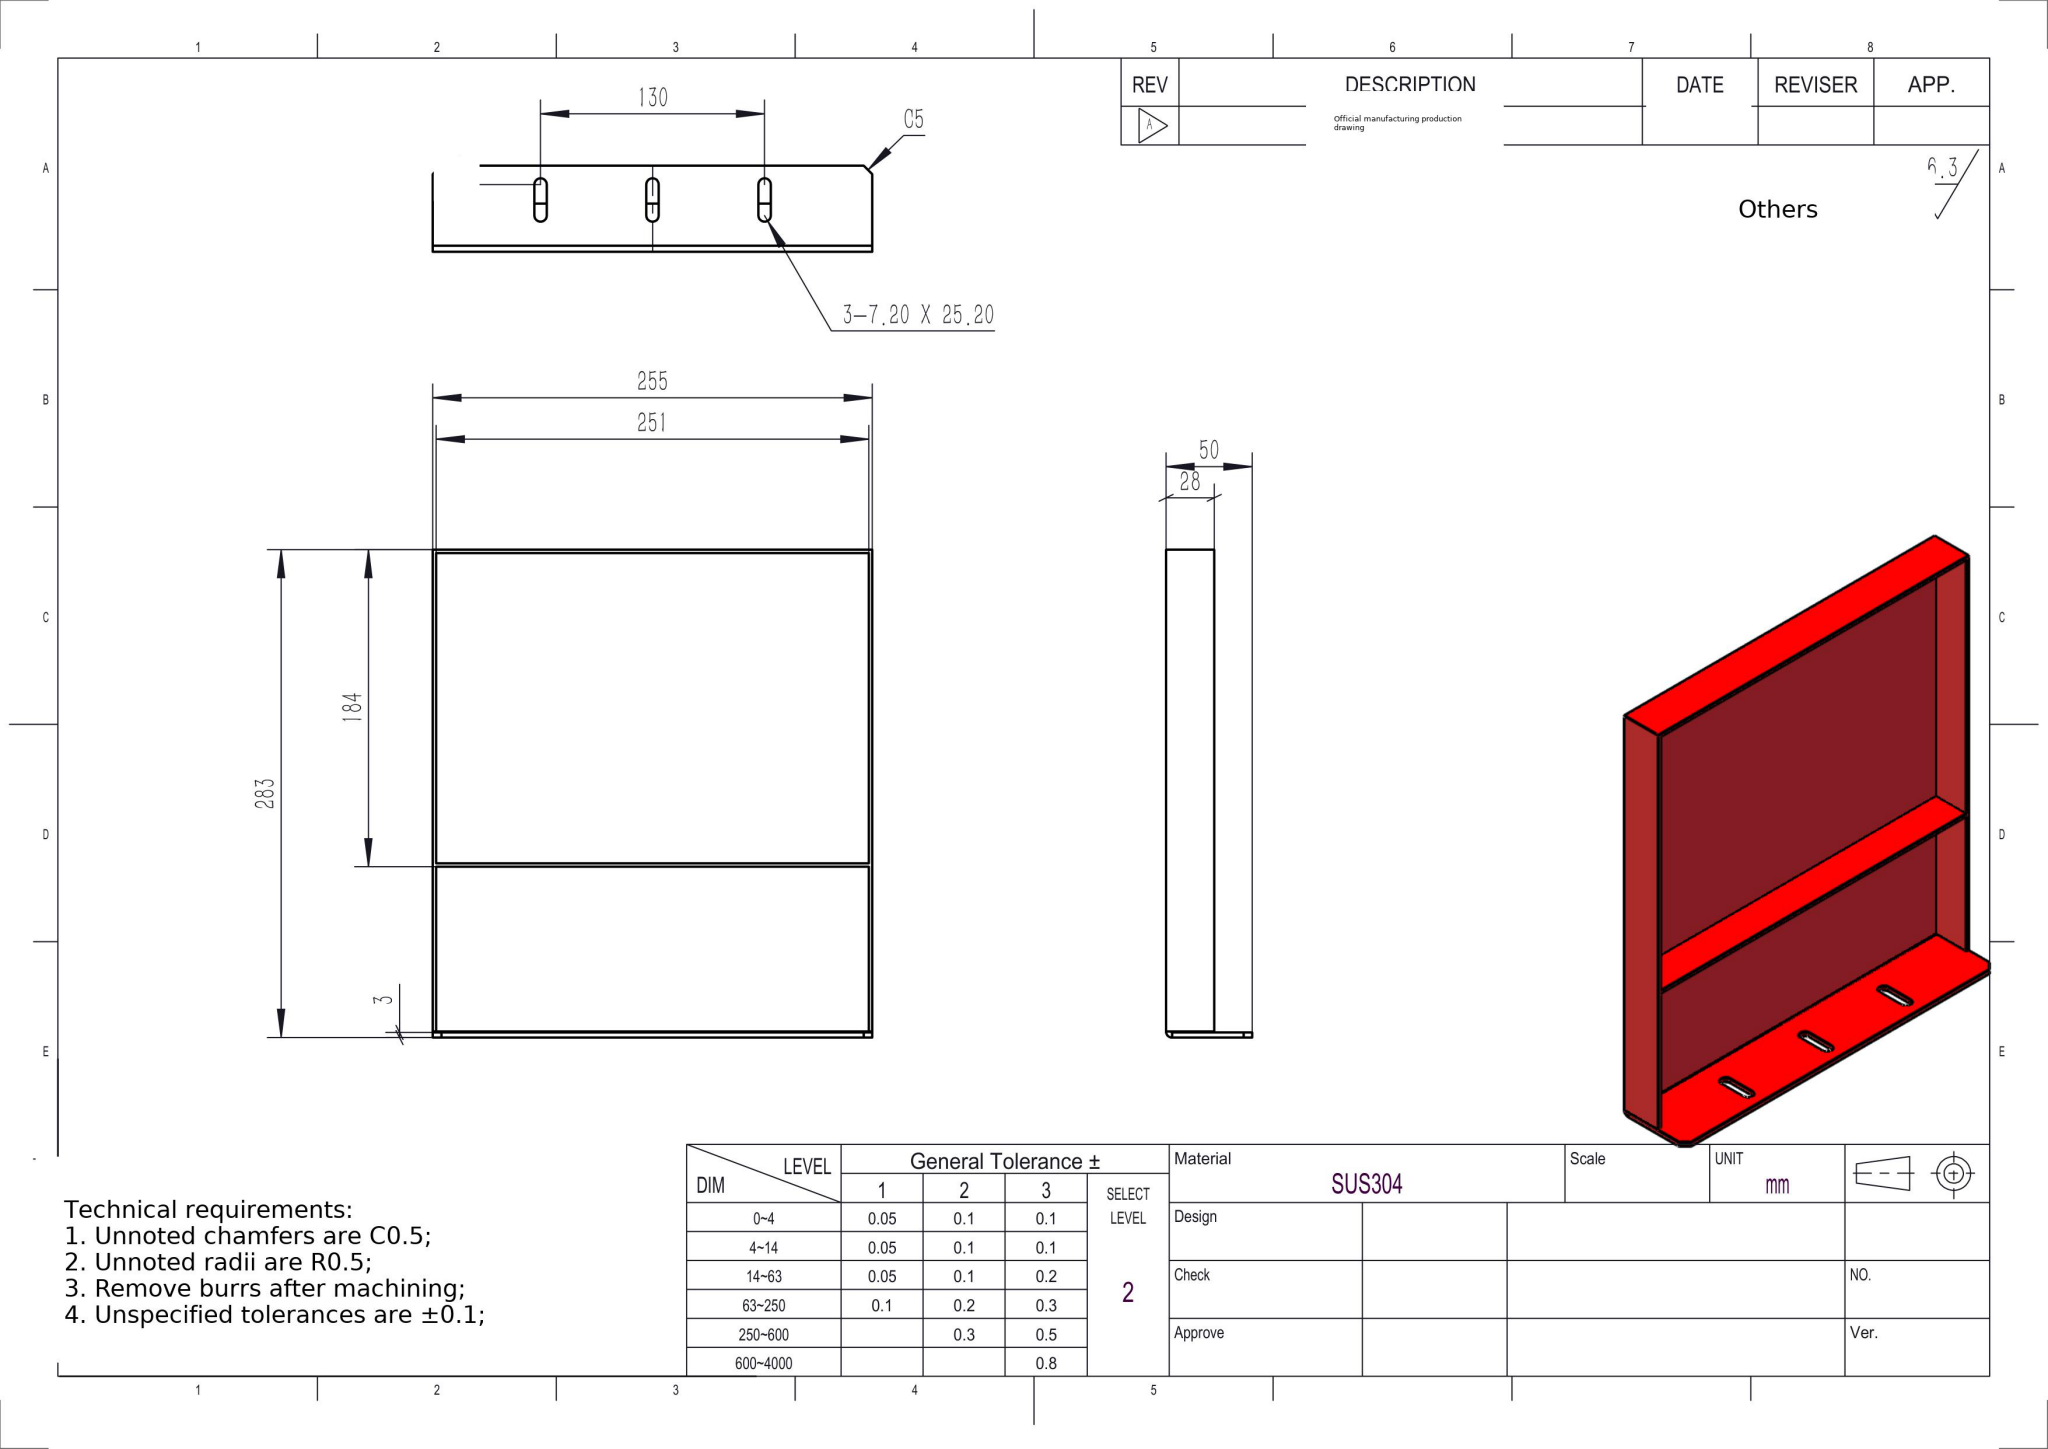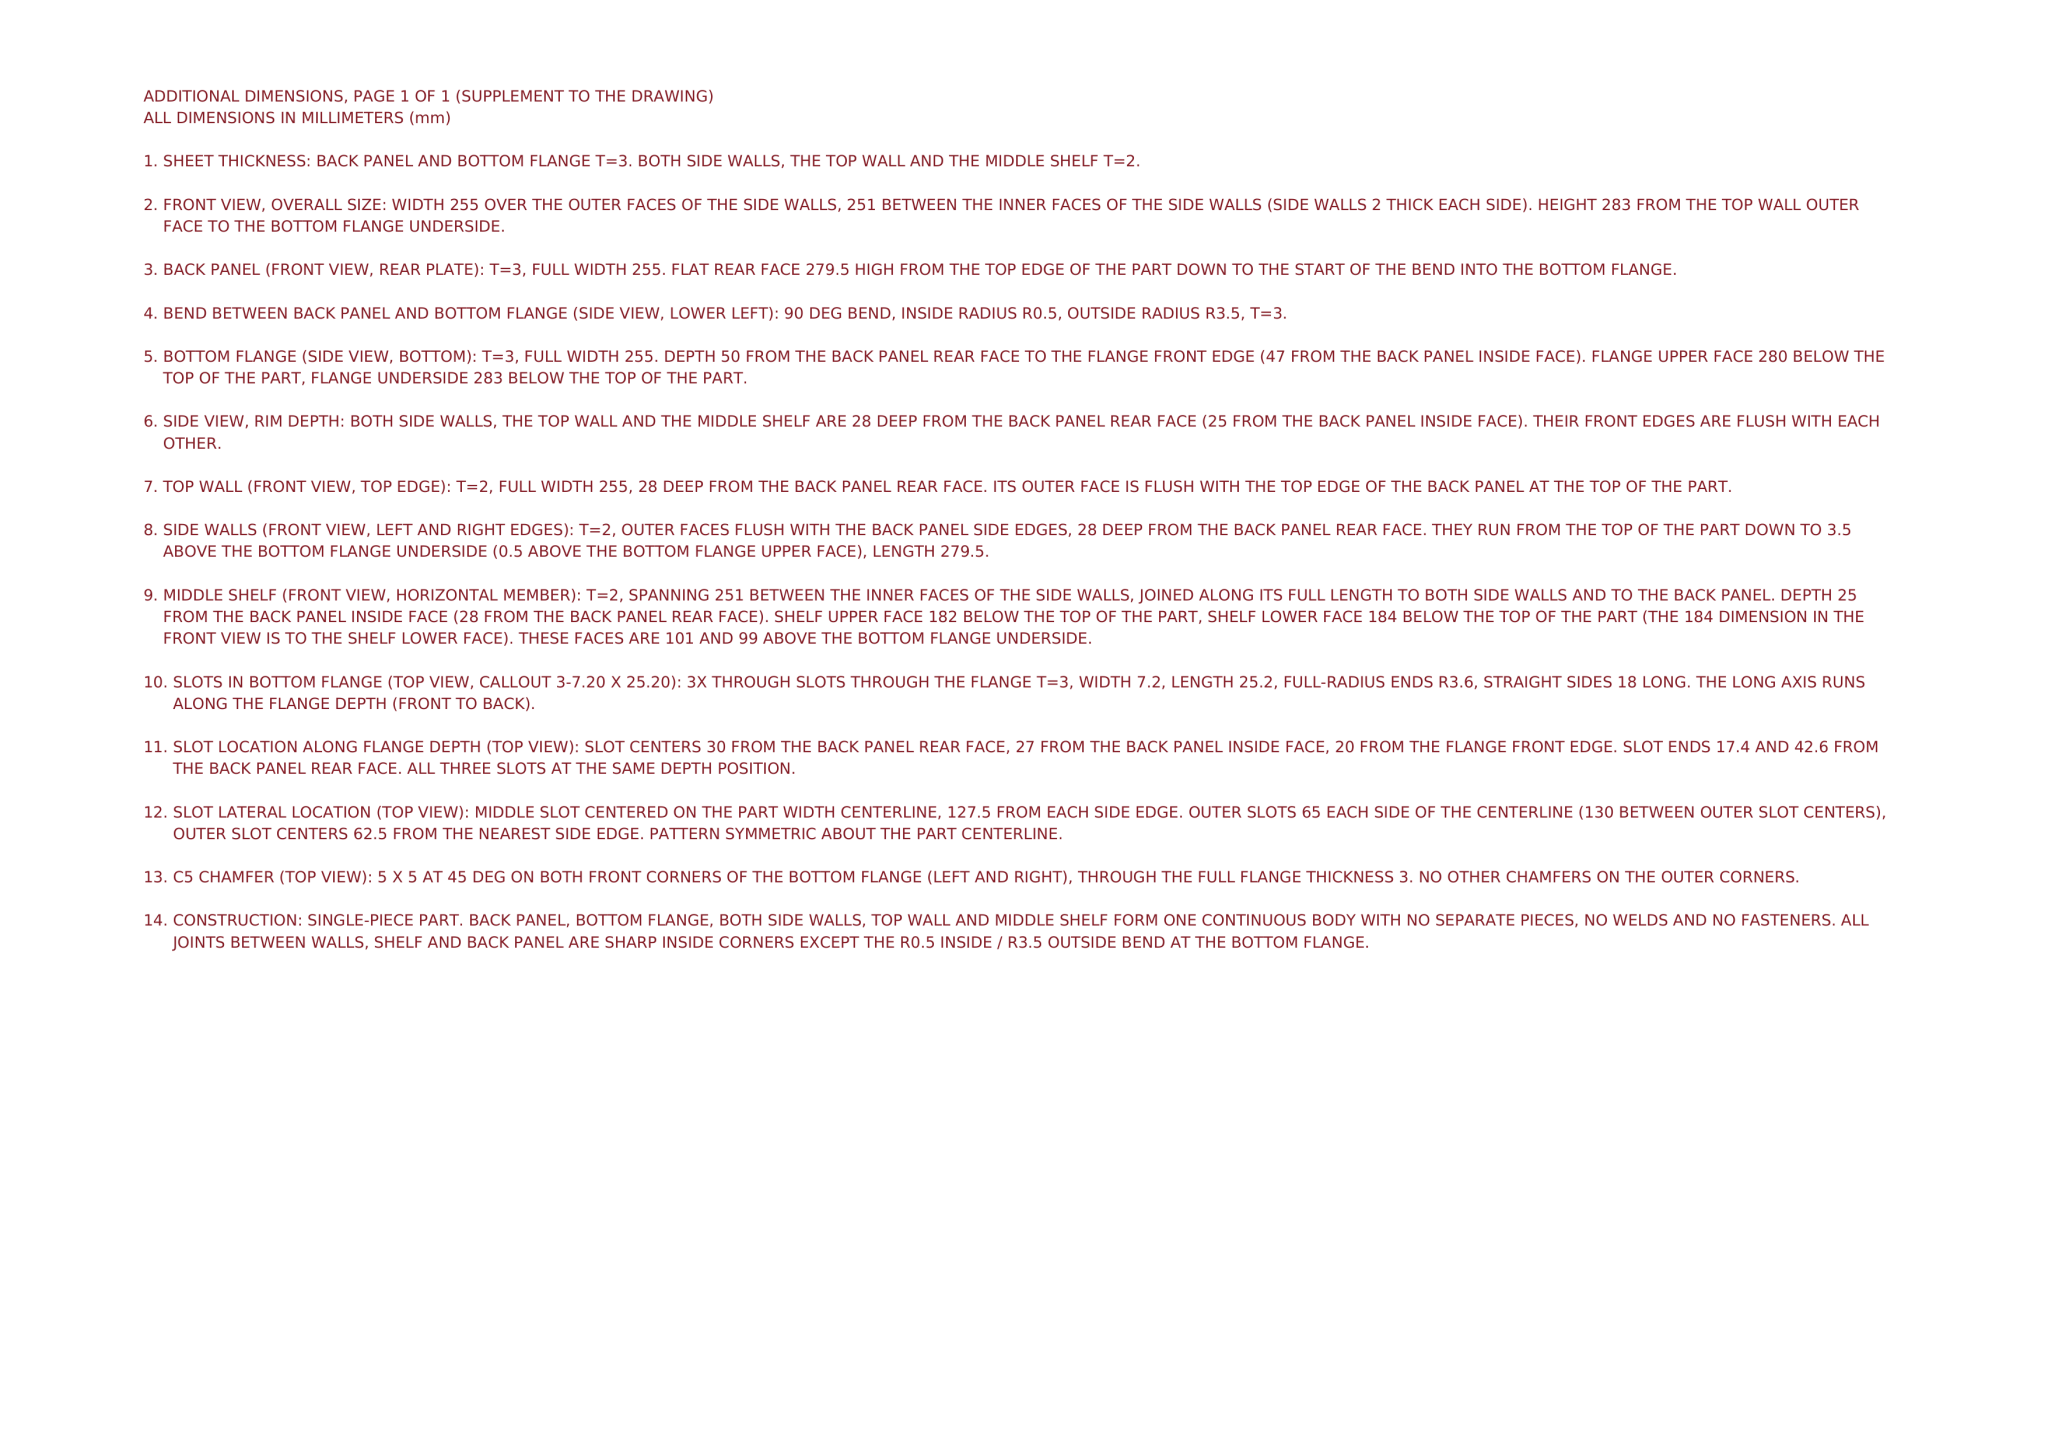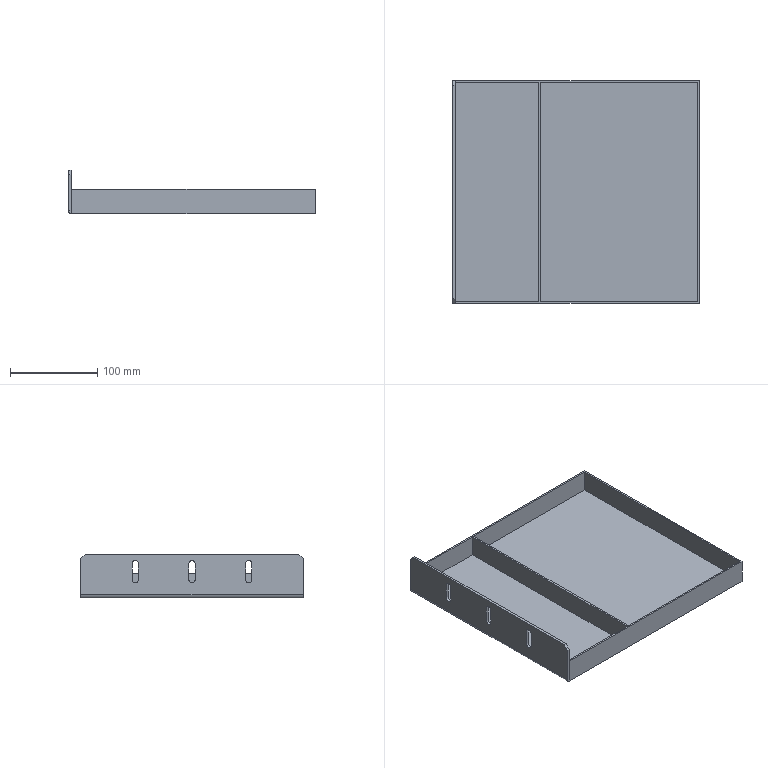Part | NX | mm | 1 solid | 42 faces | box 283 x 255 x 50 mm | volume 303235 mm3 | plane 31 | cylinder 11 | commonest cylinder face diameters 7.2 x9 7 x1 1 x1